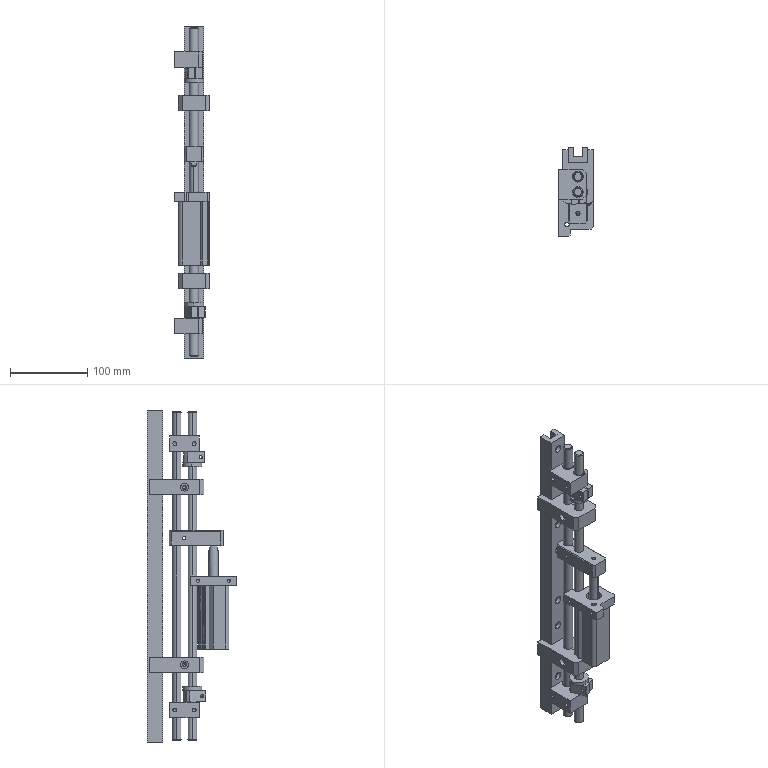Assembly | SolidWorks | mm | 21 component files | 21 solids | 521 faces | box 45 x 115.5 x 430 mm | volume 517809 mm3 | plane 233 | cylinder 220 | cone 68 | commonest cylinder face diameters 12 x40 5.5 x32 10 x26 4.2 x18 14 x16 4.26 x10 5 x8 25 x8
Bill of materials:
50 | 2 |  | Long, thin solid cylindrical rod or pin with plain ends that appear to be chamfered.
51 | 2 |  | Rectangular block with two parallel round through-holes in the top face and two chamfered vertical corners on one side.
52 | 1 |  | Flat plate, roughly T- or cross-shaped, with a large central through-hole, two smaller through-holes at diagonally opposite corners, rounded inside corners at the notches, and chamfered outer corners.
53 | 4 |  | Short, thin-walled cylindrical tube or sleeve with open ends and small chamfers on the end edges.
54 | 1 |  | Long, straight channel-section bar (U/C profile) with a row of small round holes spaced along its length on one face.
55 | 2 |  | Rectangular block with an open rectangular U-slot at one end, two round through-holes joined by a narrow slit, and chamfered corners at the opposite end.
56 | 1 |  | Rectangular bar-shaped block with chamfered corners and edges, two larger vertical through-holes joined by a narrow slit, a smaller vertical through-hole near one end, and a horizontal cross-hole through a side face.
57 | 2 |  | Split-clamp-style block with a large through-bore, a straight slit from the bore to the outer edge, a stepped (counterbored-looking) cross-hole perpendicular to the slit, and chamfered edges and corners.
58 | 2 |  | Flat circular ring, washer- or spacer-like, with a concentric through-hole and plain square edges.
Mates:
1. coincident | 54-1 face at (-12.5, 20, 430) dir (-1, 0, 0) | 55-1 face at (-12.5, 27, 130) dir (1, 0, 0)
2. concentric | 54-1 face at (0, 8, 100) dir (0, 1, 0) r 5 | 55-1 face at (0, 0, 100) dir (0, 1, 0) r 2.1
3. coincident | 54-1 face at (12.5, 0, 430) dir (0, -1, 0) | 55-1 face at (12.5, 0, 130) dir (0, 1, 0)
4. concentric | 54-1 face at (0, 8, 330) dir (0, 1, 0) r 2.75 | 55-2 face at (0, 0, 330) dir (0, 1, 0) r 2.1
5. coincident | 54-1 face at (12.5, 0, 430) dir (0, -1, 0) | 55-2 face at (12.5, 0, 360) dir (0, 1, 0)
6. concentric | 55-2 face at (0, -18, 360) dir (0, 0, -1) r 6 | 50-1 face at (0, -18, 427.5) dir (0, 0, 1) r 6
7. width | 55-1 face at (-20, 27, 90) dir (0, 0, -1) | 55-2 face at (-20, 27, 340) dir (0, 0, 1) | 50-1 face at (0, -18, 427.5) dir (0, 0, 1) | 50-1 face at (0, -18, 2.5) dir (0, 0, -1)
8. concentric | 55-2 face at (0, -38, 360) dir (0, 0, -1) r 6 | 50-2 face at (0, -38, 427.5) dir (0, 0, 1) r 6
9. coincident | 50-1 face at (0, -18, 2.5) dir (0, 0, -1) | 50-2 face at (0, -38, 2.5) dir (0, 0, -1)
10. concentric | 50-1 face at (0, -18, 427.5) dir (0, 0, 1) r 6 | 56-1 face at (0, -18, 273.966) dir (0, 0, -1) r 6
11. concentric | 50-2 face at (0, -38, 427.5) dir (0, 0, 1) r 6 | 51-1 face at (0, -38, 376.398) dir (0, 0, 1) r 7
12. concentric | 50-1 face at (0, -18, 427.5) dir (0, 0, 1) r 6 | 51-1 face at (0, -18, 376.398) dir (0, 0, 1) r 7
13. concentric | 50-2 face at (0, -38, 427.5) dir (0, 0, 1) r 6 | 53-1 face at (0, -38, 376.398) dir (0, 0, -1) r 6
14. coincident | 51-1 face at (-7, -28, 376.398) dir (0, 0, -1) | 53-1 face at (6, -38, 376.398) dir (0, 0, -1)
15. concentric | 50-1 face at (0, -18, 427.5) dir (0, 0, 1) r 6 | 53-2 face at (0, -18, 376.398) dir (0, 0, -1) r 6
16. coincident | 51-1 face at (-7, -28, 376.398) dir (0, 0, -1) | 53-2 face at (6, -18, 376.398) dir (0, 0, -1)
17. concentric | 50-2 face at (0, -38, 427.5) dir (0, 0, 1) r 6 | 56-1 face at (0, -38, 273.966) dir (0, 0, -1) r 6
18. concentric | 50-2 face at (0, -38, 427.5) dir (0, 0, 1) r 6 | 57-1 face at (0, -38, 66.954) dir (0, 0, -1) r 6
19. concentric | 50-2 face at (0, -38, 427.5) dir (0, 0, 1) r 6 | 58-1 face at (0, -38, 66.954) dir (0, 0, -1) r 6
20. coincident | 57-1 face at (0, -38, 66.954) dir (0, 0, 1) | 58-1 face at (6, -38, 66.954) dir (0, 0, -1)
21. concentric | 50-2 face at (0, -38, 427.5) dir (0, 0, 1) r 6 | 58-2 face at (0, -38, 356.398) dir (0, 0, -1) r 6
22. concentric | 50-2 face at (0, -38, 427.5) dir (0, 0, 1) r 6 | 57-2 face at (0, -38, 376.398) dir (0, 0, -1) r 6
23. coincident | 58-2 face at (0.3059, -32.008, 361.398) dir (0, 0, 1) | 57-2 face at (0, -38, 361.398) dir (0, 0, -1)
24. concentric | 50-1 face at (0, -18, 427.5) dir (0, 0, 1) r 6 | 51-2 face at (0, -18, 31.394) dir (0, 0, 1) r 7
25. concentric | 50-2 face at (0, -38, 427.5) dir (0, 0, 1) r 6 | 51-2 face at (0, -38, 31.394) dir (0, 0, 1) r 7
26. concentric | 50-2 face at (0, -38, 427.5) dir (0, 0, 1) r 6 | 53-3 face at (0, -38, 31.394) dir (0, 0, -1) r 7
27. coincident | 51-2 face at (-7, -28, 31.394) dir (0, 0, -1) | 53-3 face at (6, -38, 31.394) dir (0, 0, -1)
28. concentric | 50-1 face at (0, -18, 427.5) dir (0, 0, 1) r 6 | 53-4 face at (0, -18, 31.394) dir (0, 0, -1) r 7
29. coincident | 51-2 face at (-7, -28, 31.394) dir (0, 0, -1) | 53-4 face at (6, -18, 31.394) dir (0, 0, -1)
30. distance | 51-1 face at (-7, -28, 396.398) dir (0, 0, 1) | 50-2 face at (0, -38, 427.5) dir (0, 0, 1)
31. distance | 56-1 face at (0, -38, 273.966) dir (0, 0, 1) | 55-2 face at (-20, 27, 320) dir (0, 0, -1)
32. concentric | 52-1 face at (14.142, -51.358, 214.893) dir (0, 0, -1) r 3.15 | CDQ2B25-50DZ-M9N(0_0_0)-1/CDQ2B25-50-M9N(0_0)_BODY-1 face at (14.142, -51.358, 120.393) dir (0, 0, 1) r 4.5
33. concentric | 52-1 face at (-14.142, -79.642, 214.893) dir (0, 0, -1) r 3.15 | CDQ2B25-50DZ-M9N(0_0_0)-1/CDQ2B25-50-M9N(0_0)_BODY-1 face at (-14.142, -79.642, 120.393) dir (0, 0, 1) r 4.5
34. coincident | 52-1 face at (0, -65.5, 202.893) dir (0, 0, -1) | CDQ2B25-50DZ-M9N(0_0_0)-1/CDQ2B25-50-M9N(0_0)_BODY-1 face at (-14.142, -79.642, 202.893) dir (0, 0, 1)
35. coincident | 51-1 face at (-7, -28, 376.398) dir (0, 0, -1) | 57-2 face at (0, -38, 376.398) dir (0, 0, 1)
36. coincident | 56-1 face at (0, -38, 253.966) dir (0, 0, -1) | CDQ2B25-50DZ-M9N(0_0_0)-1/CDQ2B25-50M9N(0_0)_CYROD-1 face at (3, -65.5, 253.966) dir (0, 0, 1)
37. coincident | CDQ2B25-50-M9N(0_0)_BODY-1 axis at (-80.9, 0, 0) dir (1, 0, 0) | CDQ2B25-50M9N(0_0)_CYROD-1 axis at (30.9, 0, 0) dir (-1, 0, 0)
38. angle | CDQ2B25-50M9N(0_0)_CYROD-1 plane at (-50, 0, 0) dir (0, 0, -1) | CDQ2B25-50-M9N(0_0)_BODY-1 plane at (0, 0, 0) dir (0, 0, -1)
39. coincident | CDQ2B25-50-M9N(0_0)_BODY-1 axis at (80.9, -10.748, -14.708) dir (-1, 0, 0) | D_M9N(CQ2_25)-1 axis at (-71.4, -10.748, -14.708) dir (1, 0, 0)
40. distance | D_M9N(CQ2_25)-2 plane at (74.5, -14.708, -10.748) dir (1, 0, 0) | CDQ2B25-50-M9N(0_0)_BODY-1 plane at (82.5, 0, 0) dir (-1, 0, 0)
41. coincident | CDQ2B25-50-M9N(0_0)_BODY-1 axis at (-80.9, -14.708, -10.748) dir (1, 0, 0) | D_M9N(CQ2_25)-2 axis at (155.4, -14.708, -10.748) dir (-1, 0, 0)
42. angle | D_M9N(CQ2_25)-2 plane at (74.5, -14.708, -10.748) dir (0, 0.7071, -0.7071) | CDQ2B25-50-M9N(0_0)_BODY-1 plane at (0, 0, -10.748) dir (0, 0, -1)
43. distance | CDQ2B25-50M9N(0_0)_CYROD-1 face at (15, 12.5, 0) dir (1, 0, 0) | CDQ2B25-50-M9N(0_0)_BODY-1 face at (65, 12.5, 0) dir (-1, 0, 0)